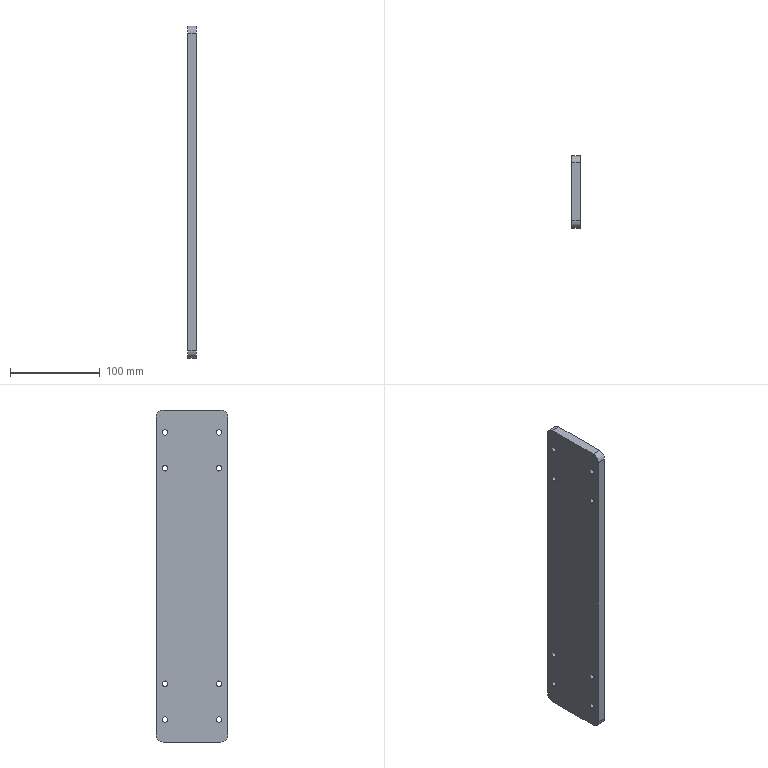Component | SolidWorks | VerticalMovingRectangularTubeWeldment-1_RectangularTubeEndPlate-2 | 1 solid | 26 faces | box 10 x 80 x 370 mm | volume 293189 mm3 | cylinder 20 | plane 6 | commonest cylinder face diameters 6 x16 16 x4 | material Plain Carbon Steel
STEP:
#1=COLOUR_RGB('',0.7922,0.8196,0.9333);
#2=FILL_AREA_STYLE_COLOUR('',#1);
#3=FILL_AREA_STYLE('',(#2));
#4=SURFACE_STYLE_FILL_AREA(#3);
#5=SURFACE_SIDE_STYLE('',(#4));
#6=SURFACE_STYLE_USAGE(.BOTH.,#5);
#7=PRESENTATION_STYLE_ASSIGNMENT((#6));
#8=CARTESIAN_POINT('',(19.685,1.181,12.913));
#9=VERTEX_POINT('',#8);
#10=CARTESIAN_POINT('',(19.685,1.181,12.677));
#11=VERTEX_POINT('',#10);
#12=CARTESIAN_POINT('',(19.685,1.181,12.795));
#13=DIRECTION('',(1.,0.,0.));
#14=DIRECTION('',(0.,1.,0.));
#15=AXIS2_PLACEMENT_3D('',#12,#13,#14);
#16=CIRCLE('',#15,0.1181);
#17=EDGE_CURVE('',#9,#11,#16,.T.);
#18=ORIENTED_EDGE('',*,*,#17,.F.);
#19=CARTESIAN_POINT('',(20.079,1.181,12.913));
#20=VERTEX_POINT('',#19);
#21=CARTESIAN_POINT('',(20.079,1.181,12.913));
#22=DIRECTION('',(1.,0.,0.));
#23=VECTOR('',#22,39.37);
#24=LINE('',#21,#23);
#25=EDGE_CURVE('',#9,#20,#24,.T.);
#26=ORIENTED_EDGE('',*,*,#25,.T.);
#27=CARTESIAN_POINT('',(20.079,1.181,12.677));
#28=VERTEX_POINT('',#27);
#29=CARTESIAN_POINT('',(20.079,1.181,12.795));
#30=DIRECTION('',(1.,0.,0.));
#31=DIRECTION('',(0.,0.,-1.));
#32=AXIS2_PLACEMENT_3D('',#29,#30,#31);
#33=CIRCLE('',#32,0.1181);
#34=EDGE_CURVE('',#20,#28,#33,.T.);
#35=ORIENTED_EDGE('',*,*,#34,.T.);
#36=CARTESIAN_POINT('',(20.079,1.181,12.677));
#37=DIRECTION('',(1.,0.,0.));
#38=VECTOR('',#37,39.37);
#39=LINE('',#36,#38);
#40=EDGE_CURVE('',#11,#28,#39,.T.);
#41=ORIENTED_EDGE('',*,*,#40,.F.);
#42=EDGE_LOOP('',(#18,#26,#35,#41));
#43=FACE_OUTER_BOUND('',#42,.T.);
#44=CARTESIAN_POINT('',(20.079,1.181,12.795));
#45=DIRECTION('',(1.,0.,0.));
#46=DIRECTION('',(0.,0.,-1.));
#47=AXIS2_PLACEMENT_3D('',#44,#45,#46);
#48=CYLINDRICAL_SURFACE('',#47,0.1181);
#49=ADVANCED_FACE('',(#43),#48,.F.);
#50=CARTESIAN_POINT('',(19.685,1.181,11.339));
#51=VERTEX_POINT('',#50);
#52=CARTESIAN_POINT('',(19.685,1.181,11.102));
#53=VERTEX_POINT('',#52);
#54=CARTESIAN_POINT('',(19.685,1.181,11.22));
#55=DIRECTION('',(1.,0.,0.));
#56=DIRECTION('',(0.,1.,0.));
#57=AXIS2_PLACEMENT_3D('',#54,#55,#56);
#58=CIRCLE('',#57,0.1181);
#59=EDGE_CURVE('',#51,#53,#58,.T.);
#60=ORIENTED_EDGE('',*,*,#59,.F.);
#61=CARTESIAN_POINT('',(20.079,1.181,11.339));
#62=VERTEX_POINT('',#61);
#63=CARTESIAN_POINT('',(20.079,1.181,11.339));
#64=DIRECTION('',(1.,0.,0.));
#65=VECTOR('',#64,39.37);
#66=LINE('',#63,#65);
#67=EDGE_CURVE('',#51,#62,#66,.T.);
#68=ORIENTED_EDGE('',*,*,#67,.T.);
#69=CARTESIAN_POINT('',(20.079,1.181,11.102));
#70=VERTEX_POINT('',#69);
#71=CARTESIAN_POINT('',(20.079,1.181,11.22));
#72=DIRECTION('',(1.,0.,0.));
#73=DIRECTION('',(0.,0.,-1.));
#74=AXIS2_PLACEMENT_3D('',#71,#72,#73);
#75=CIRCLE('',#74,0.1181);
#76=EDGE_CURVE('',#62,#70,#75,.T.);
#77=ORIENTED_EDGE('',*,*,#76,.T.);
#78=CARTESIAN_POINT('',(20.079,1.181,11.102));
#79=DIRECTION('',(1.,0.,0.));
#80=VECTOR('',#79,39.37);
#81=LINE('',#78,#80);
#82=EDGE_CURVE('',#53,#70,#81,.T.);
#83=ORIENTED_EDGE('',*,*,#82,.F.);
#84=EDGE_LOOP('',(#60,#68,#77,#83));
#85=FACE_OUTER_BOUND('',#84,.T.);
#86=CARTESIAN_POINT('',(20.079,1.181,11.22));
#87=DIRECTION('',(1.,0.,0.));
#88=DIRECTION('',(0.,0.,-1.));
#89=AXIS2_PLACEMENT_3D('',#86,#87,#88);
#90=CYLINDRICAL_SURFACE('',#89,0.1181);
#91=ADVANCED_FACE('',(#85),#90,.F.);
#92=CARTESIAN_POINT('',(19.685,1.181,1.89));
#93=VERTEX_POINT('',#92);
#94=CARTESIAN_POINT('',(19.685,1.181,1.654));
#95=VERTEX_POINT('',#94);
#96=CARTESIAN_POINT('',(19.685,1.181,1.772));
#97=DIRECTION('',(1.,0.,0.));
#98=DIRECTION('',(0.,1.,0.));
#99=AXIS2_PLACEMENT_3D('',#96,#97,#98);
#100=CIRCLE('',#99,0.1181);
#101=EDGE_CURVE('',#93,#95,#100,.T.);
#102=ORIENTED_EDGE('',*,*,#101,.F.);
#103=CARTESIAN_POINT('',(20.079,1.181,1.89));
#104=VERTEX_POINT('',#103);
#105=CARTESIAN_POINT('',(20.079,1.181,1.89));
#106=DIRECTION('',(1.,0.,0.));
#107=VECTOR('',#106,39.37);
#108=LINE('',#105,#107);
#109=EDGE_CURVE('',#93,#104,#108,.T.);
#110=ORIENTED_EDGE('',*,*,#109,.T.);
#111=CARTESIAN_POINT('',(20.079,1.181,1.654));
#112=VERTEX_POINT('',#111);
#113=CARTESIAN_POINT('',(20.079,1.181,1.772));
#114=DIRECTION('',(1.,0.,0.));
#115=DIRECTION('',(0.,0.,-1.));
#116=AXIS2_PLACEMENT_3D('',#113,#114,#115);
#117=CIRCLE('',#116,0.1181);
#118=EDGE_CURVE('',#104,#112,#117,.T.);
#119=ORIENTED_EDGE('',*,*,#118,.T.);
#120=CARTESIAN_POINT('',(20.079,1.181,1.654));
#121=DIRECTION('',(1.,0.,0.));
#122=VECTOR('',#121,39.37);
#123=LINE('',#120,#122);
#124=EDGE_CURVE('',#95,#112,#123,.T.);
#125=ORIENTED_EDGE('',*,*,#124,.F.);
#126=EDGE_LOOP('',(#102,#110,#119,#125));
#127=FACE_OUTER_BOUND('',#126,.T.);
#128=CARTESIAN_POINT('',(20.079,1.181,1.772));
#129=DIRECTION('',(1.,0.,0.));
#130=DIRECTION('',(0.,0.,-1.));
#131=AXIS2_PLACEMENT_3D('',#128,#129,#130);
#132=CYLINDRICAL_SURFACE('',#131,0.1181);
#133=ADVANCED_FACE('',(#127),#132,.F.);
#134=CARTESIAN_POINT('',(19.685,1.181,0.315));
#135=VERTEX_POINT('',#134);
#136=CARTESIAN_POINT('',(19.685,1.181,0.07874));
#137=VERTEX_POINT('',#136);
#138=CARTESIAN_POINT('',(19.685,1.181,0.1969));
#139=DIRECTION('',(1.,0.,0.));
#140=DIRECTION('',(0.,1.,-0.));
#141=AXIS2_PLACEMENT_3D('',#138,#139,#140);
#142=CIRCLE('',#141,0.1181);
#143=EDGE_CURVE('',#135,#137,#142,.T.);
#144=ORIENTED_EDGE('',*,*,#143,.F.);
#145=CARTESIAN_POINT('',(20.079,1.181,0.315));
#146=VERTEX_POINT('',#145);
#147=CARTESIAN_POINT('',(20.079,1.181,0.315));
#148=DIRECTION('',(1.,0.,0.));
#149=VECTOR('',#148,39.37);
#150=LINE('',#147,#149);
#151=EDGE_CURVE('',#135,#146,#150,.T.);
#152=ORIENTED_EDGE('',*,*,#151,.T.);
#153=CARTESIAN_POINT('',(20.079,1.181,0.07874));
#154=VERTEX_POINT('',#153);
#155=CARTESIAN_POINT('',(20.079,1.181,0.1969));
#156=DIRECTION('',(1.,0.,0.));
#157=DIRECTION('',(0.,0.,-1.));
#158=AXIS2_PLACEMENT_3D('',#155,#156,#157);
#159=CIRCLE('',#158,0.1181);
#160=EDGE_CURVE('',#146,#154,#159,.T.);
#161=ORIENTED_EDGE('',*,*,#160,.T.);
#162=CARTESIAN_POINT('',(20.079,1.181,0.07874));
#163=DIRECTION('',(1.,0.,0.));
#164=VECTOR('',#163,39.37);
#165=LINE('',#162,#164);
#166=EDGE_CURVE('',#137,#154,#165,.T.);
#167=ORIENTED_EDGE('',*,*,#166,.F.);
#168=EDGE_LOOP('',(#144,#152,#161,#167));
#169=FACE_OUTER_BOUND('',#168,.T.);
#170=CARTESIAN_POINT('',(20.079,1.181,0.1969));
#171=DIRECTION('',(1.,0.,0.));
#172=DIRECTION('',(0.,0.,-1.));
#173=AXIS2_PLACEMENT_3D('',#170,#171,#172);
#174=CYLINDRICAL_SURFACE('',#173,0.1181);
#175=ADVANCED_FACE('',(#169),#174,.F.);
#176=CARTESIAN_POINT('',(19.685,-1.181,12.913));
#177=VERTEX_POINT('',#176);
#178=CARTESIAN_POINT('',(19.685,-1.181,12.677));
#179=VERTEX_POINT('',#178);
#180=CARTESIAN_POINT('',(19.685,-1.181,12.795));
#181=DIRECTION('',(1.,0.,0.));
#182=DIRECTION('',(0.,1.,0.));
#183=AXIS2_PLACEMENT_3D('',#180,#181,#182);
#184=CIRCLE('',#183,0.1181);
#185=EDGE_CURVE('',#177,#179,#184,.T.);
#186=ORIENTED_EDGE('',*,*,#185,.F.);
#187=CARTESIAN_POINT('',(20.079,-1.181,12.913));
#188=VERTEX_POINT('',#187);
#189=CARTESIAN_POINT('',(20.079,-1.181,12.913));
#190=DIRECTION('',(1.,0.,0.));
#191=VECTOR('',#190,39.37);
#192=LINE('',#189,#191);
#193=EDGE_CURVE('',#177,#188,#192,.T.);
#194=ORIENTED_EDGE('',*,*,#193,.T.);
#195=CARTESIAN_POINT('',(20.079,-1.181,12.677));
#196=VERTEX_POINT('',#195);
#197=CARTESIAN_POINT('',(20.079,-1.181,12.795));
#198=DIRECTION('',(1.,0.,0.));
#199=DIRECTION('',(0.,0.,-1.));
#200=AXIS2_PLACEMENT_3D('',#197,#198,#199);
#201=CIRCLE('',#200,0.1181);
#202=EDGE_CURVE('',#188,#196,#201,.T.);
#203=ORIENTED_EDGE('',*,*,#202,.T.);
#204=CARTESIAN_POINT('',(20.079,-1.181,12.677));
#205=DIRECTION('',(1.,0.,0.));
#206=VECTOR('',#205,39.37);
#207=LINE('',#204,#206);
#208=EDGE_CURVE('',#179,#196,#207,.T.);
#209=ORIENTED_EDGE('',*,*,#208,.F.);
#210=EDGE_LOOP('',(#186,#194,#203,#209));
#211=FACE_OUTER_BOUND('',#210,.T.);
#212=CARTESIAN_POINT('',(20.079,-1.181,12.795));
#213=DIRECTION('',(1.,0.,0.));
#214=DIRECTION('',(0.,0.,-1.));
#215=AXIS2_PLACEMENT_3D('',#212,#213,#214);
#216=CYLINDRICAL_SURFACE('',#215,0.1181);
#217=ADVANCED_FACE('',(#211),#216,.F.);
#218=CARTESIAN_POINT('',(19.685,-1.181,11.339));
#219=VERTEX_POINT('',#218);
#220=CARTESIAN_POINT('',(19.685,-1.181,11.102));
#221=VERTEX_POINT('',#220);
#222=CARTESIAN_POINT('',(19.685,-1.181,11.22));
#223=DIRECTION('',(1.,0.,0.));
#224=DIRECTION('',(0.,1.,0.));
#225=AXIS2_PLACEMENT_3D('',#222,#223,#224);
#226=CIRCLE('',#225,0.1181);
#227=EDGE_CURVE('',#219,#221,#226,.T.);
#228=ORIENTED_EDGE('',*,*,#227,.F.);
#229=CARTESIAN_POINT('',(20.079,-1.181,11.339));
#230=VERTEX_POINT('',#229);
#231=CARTESIAN_POINT('',(20.079,-1.181,11.339));
#232=DIRECTION('',(1.,0.,0.));
#233=VECTOR('',#232,39.37);
#234=LINE('',#231,#233);
#235=EDGE_CURVE('',#219,#230,#234,.T.);
#236=ORIENTED_EDGE('',*,*,#235,.T.);
#237=CARTESIAN_POINT('',(20.079,-1.181,11.102));
#238=VERTEX_POINT('',#237);
#239=CARTESIAN_POINT('',(20.079,-1.181,11.22));
#240=DIRECTION('',(1.,0.,0.));
#241=DIRECTION('',(0.,0.,-1.));
#242=AXIS2_PLACEMENT_3D('',#239,#240,#241);
#243=CIRCLE('',#242,0.1181);
#244=EDGE_CURVE('',#230,#238,#243,.T.);
#245=ORIENTED_EDGE('',*,*,#244,.T.);
#246=CARTESIAN_POINT('',(20.079,-1.181,11.102));
#247=DIRECTION('',(1.,0.,0.));
#248=VECTOR('',#247,39.37);
#249=LINE('',#246,#248);
#250=EDGE_CURVE('',#221,#238,#249,.T.);
#251=ORIENTED_EDGE('',*,*,#250,.F.);
#252=EDGE_LOOP('',(#228,#236,#245,#251));
#253=FACE_OUTER_BOUND('',#252,.T.);
#254=CARTESIAN_POINT('',(20.079,-1.181,11.22));
#255=DIRECTION('',(1.,0.,0.));
#256=DIRECTION('',(0.,0.,-1.));
#257=AXIS2_PLACEMENT_3D('',#254,#255,#256);
#258=CYLINDRICAL_SURFACE('',#257,0.1181);
#259=ADVANCED_FACE('',(#253),#258,.F.);
#260=CARTESIAN_POINT('',(19.685,-1.181,1.89));
#261=VERTEX_POINT('',#260);
#262=CARTESIAN_POINT('',(19.685,-1.181,1.654));
#263=VERTEX_POINT('',#262);
#264=CARTESIAN_POINT('',(19.685,-1.181,1.772));
#265=DIRECTION('',(1.,0.,0.));
#266=DIRECTION('',(0.,1.,0.));
#267=AXIS2_PLACEMENT_3D('',#264,#265,#266);
#268=CIRCLE('',#267,0.1181);
#269=EDGE_CURVE('',#261,#263,#268,.T.);
#270=ORIENTED_EDGE('',*,*,#269,.F.);
#271=CARTESIAN_POINT('',(20.079,-1.181,1.89));
#272=VERTEX_POINT('',#271);
#273=CARTESIAN_POINT('',(20.079,-1.181,1.89));
#274=DIRECTION('',(1.,0.,0.));
#275=VECTOR('',#274,39.37);
#276=LINE('',#273,#275);
#277=EDGE_CURVE('',#261,#272,#276,.T.);
#278=ORIENTED_EDGE('',*,*,#277,.T.);
#279=CARTESIAN_POINT('',(20.079,-1.181,1.654));
#280=VERTEX_POINT('',#279);
#281=CARTESIAN_POINT('',(20.079,-1.181,1.772));
#282=DIRECTION('',(1.,0.,0.));
#283=DIRECTION('',(0.,0.,-1.));
#284=AXIS2_PLACEMENT_3D('',#281,#282,#283);
#285=CIRCLE('',#284,0.1181);
#286=EDGE_CURVE('',#272,#280,#285,.T.);
#287=ORIENTED_EDGE('',*,*,#286,.T.);
#288=CARTESIAN_POINT('',(20.079,-1.181,1.654));
#289=DIRECTION('',(1.,0.,0.));
#290=VECTOR('',#289,39.37);
#291=LINE('',#288,#290);
#292=EDGE_CURVE('',#263,#280,#291,.T.);
#293=ORIENTED_EDGE('',*,*,#292,.F.);
#294=EDGE_LOOP('',(#270,#278,#287,#293));
#295=FACE_OUTER_BOUND('',#294,.T.);
#296=CARTESIAN_POINT('',(20.079,-1.181,1.772));
#297=DIRECTION('',(1.,0.,0.));
#298=DIRECTION('',(0.,0.,-1.));
#299=AXIS2_PLACEMENT_3D('',#296,#297,#298);
#300=CYLINDRICAL_SURFACE('',#299,0.1181);
#301=ADVANCED_FACE('',(#295),#300,.F.);
#302=CARTESIAN_POINT('',(19.685,-1.181,0.315));
#303=VERTEX_POINT('',#302);
#304=CARTESIAN_POINT('',(19.685,-1.181,0.07874));
#305=VERTEX_POINT('',#304);
#306=CARTESIAN_POINT('',(19.685,-1.181,0.1969));
#307=DIRECTION('',(1.,0.,0.));
#308=DIRECTION('',(0.,1.,-0.));
#309=AXIS2_PLACEMENT_3D('',#306,#307,#308);
#310=CIRCLE('',#309,0.1181);
#311=EDGE_CURVE('',#303,#305,#310,.T.);
#312=ORIENTED_EDGE('',*,*,#311,.F.);
#313=CARTESIAN_POINT('',(20.079,-1.181,0.315));
#314=VERTEX_POINT('',#313);
#315=CARTESIAN_POINT('',(20.079,-1.181,0.315));
#316=DIRECTION('',(1.,0.,0.));
#317=VECTOR('',#316,39.37);
#318=LINE('',#315,#317);
#319=EDGE_CURVE('',#303,#314,#318,.T.);
#320=ORIENTED_EDGE('',*,*,#319,.T.);
#321=CARTESIAN_POINT('',(20.079,-1.181,0.07874));
#322=VERTEX_POINT('',#321);
#323=CARTESIAN_POINT('',(20.079,-1.181,0.1969));
#324=DIRECTION('',(1.,0.,0.));
#325=DIRECTION('',(0.,0.,-1.));
#326=AXIS2_PLACEMENT_3D('',#323,#324,#325);
#327=CIRCLE('',#326,0.1181);
#328=EDGE_CURVE('',#314,#322,#327,.T.);
#329=ORIENTED_EDGE('',*,*,#328,.T.);
#330=CARTESIAN_POINT('',(20.079,-1.181,0.07874));
#331=DIRECTION('',(1.,0.,0.));
#332=VECTOR('',#331,39.37);
#333=LINE('',#330,#332);
#334=EDGE_CURVE('',#305,#322,#333,.T.);
#335=ORIENTED_EDGE('',*,*,#334,.F.);
#336=EDGE_LOOP('',(#312,#320,#329,#335));
#337=FACE_OUTER_BOUND('',#336,.T.);
#338=CARTESIAN_POINT('',(20.079,-1.181,0.1969));
#339=DIRECTION('',(1.,0.,0.));
#340=DIRECTION('',(0.,0.,-1.));
#341=AXIS2_PLACEMENT_3D('',#338,#339,#340);
#342=CYLINDRICAL_SURFACE('',#341,0.1181);
#343=ADVANCED_FACE('',(#337),#342,.F.);
#344=CARTESIAN_POINT('',(20.079,1.575,-0.4724));
#345=VERTEX_POINT('',#344);
#346=CARTESIAN_POINT('',(20.079,1.575,13.465));
#347=VERTEX_POINT('',#346);
#348=CARTESIAN_POINT('',(20.079,1.575,13.78));
#349=DIRECTION('',(0.,0.,1.));
#350=VECTOR('',#349,39.37);
#351=LINE('',#348,#350);
#352=EDGE_CURVE('',#345,#347,#351,.T.);
#353=ORIENTED_EDGE('',*,*,#352,.F.);
#354=CARTESIAN_POINT('',(19.685,1.575,-0.4724));
#355=VERTEX_POINT('',#354);
#356=CARTESIAN_POINT('',(20.079,1.575,-0.4724));
#357=DIRECTION('',(-1.,0.,0.));
#358=VECTOR('',#357,39.37);
#359=LINE('',#356,#358);
#360=EDGE_CURVE('',#345,#355,#359,.T.);
#361=ORIENTED_EDGE('',*,*,#360,.T.);
#362=CARTESIAN_POINT('',(19.685,1.575,13.465));
#363=VERTEX_POINT('',#362);
#364=CARTESIAN_POINT('',(19.685,1.575,13.78));
#365=DIRECTION('',(0.,0.,1.));
#366=VECTOR('',#365,39.37);
#367=LINE('',#364,#366);
#368=EDGE_CURVE('',#355,#363,#367,.T.);
#369=ORIENTED_EDGE('',*,*,#368,.T.);
#370=CARTESIAN_POINT('',(20.079,1.575,13.465));
#371=DIRECTION('',(1.,0.,0.));
#372=VECTOR('',#371,39.37);
#373=LINE('',#370,#372);
#374=EDGE_CURVE('',#363,#347,#373,.T.);
#375=ORIENTED_EDGE('',*,*,#374,.T.);
#376=EDGE_LOOP('',(#353,#361,#369,#375));
#377=FACE_OUTER_BOUND('',#376,.T.);
#378=CARTESIAN_POINT('',(20.079,1.575,13.78));
#379=DIRECTION('',(0.,-1.,0.));
#380=DIRECTION('',(0.,-0.,-1.));
#381=AXIS2_PLACEMENT_3D('',#378,#379,#380);
#382=PLANE('',#381);
#383=ADVANCED_FACE('',(#377),#382,.F.);
#384=CARTESIAN_POINT('',(19.685,1.26,13.78));
#385=VERTEX_POINT('',#384);
#386=CARTESIAN_POINT('',(19.685,-1.26,13.78));
#387=VERTEX_POINT('',#386);
#388=CARTESIAN_POINT('',(19.685,-1.575,13.78));
#389=DIRECTION('',(0.,-1.,0.));
#390=VECTOR('',#389,39.37);
#391=LINE('',#388,#390);
#392=EDGE_CURVE('',#385,#387,#391,.T.);
#393=ORIENTED_EDGE('',*,*,#392,.T.);
#394=CARTESIAN_POINT('',(20.079,-1.26,13.78));
#395=VERTEX_POINT('',#394);
#396=CARTESIAN_POINT('',(20.079,-1.26,13.78));
#397=DIRECTION('',(1.,0.,0.));
#398=VECTOR('',#397,39.37);
#399=LINE('',#396,#398);
#400=EDGE_CURVE('',#387,#395,#399,.T.);
#401=ORIENTED_EDGE('',*,*,#400,.T.);
#402=CARTESIAN_POINT('',(20.079,1.26,13.78));
#403=VERTEX_POINT('',#402);
#404=CARTESIAN_POINT('',(20.079,-1.575,13.78));
#405=DIRECTION('',(0.,-1.,0.));
#406=VECTOR('',#405,39.37);
#407=LINE('',#404,#406);
#408=EDGE_CURVE('',#403,#395,#407,.T.);
#409=ORIENTED_EDGE('',*,*,#408,.F.);
#410=CARTESIAN_POINT('',(20.079,1.26,13.78));
#411=DIRECTION('',(-1.,0.,0.));
#412=VECTOR('',#411,39.37);
#413=LINE('',#410,#412);
#414=EDGE_CURVE('',#403,#385,#413,.T.);
#415=ORIENTED_EDGE('',*,*,#414,.T.);
#416=EDGE_LOOP('',(#393,#401,#409,#415));
#417=FACE_OUTER_BOUND('',#416,.T.);
#418=CARTESIAN_POINT('',(20.079,-1.575,13.78));
#419=DIRECTION('',(0.,-0.,-1.));
#420=DIRECTION('',(-1.,0.,0.));
#421=AXIS2_PLACEMENT_3D('',#418,#419,#420);
#422=PLANE('',#421);
#423=ADVANCED_FACE('',(#417),#422,.F.);
#424=CARTESIAN_POINT('',(19.685,-1.575,13.465));
#425=VERTEX_POINT('',#424);
#426=CARTESIAN_POINT('',(19.685,-1.575,-0.4724));
#427=VERTEX_POINT('',#426);
#428=CARTESIAN_POINT('',(19.685,-1.575,13.78));
#429=DIRECTION('',(0.,-0.,-1.));
#430=VECTOR('',#429,39.37);
#431=LINE('',#428,#430);
#432=EDGE_CURVE('',#425,#427,#431,.T.);
#433=ORIENTED_EDGE('',*,*,#432,.T.);
#434=CARTESIAN_POINT('',(20.079,-1.575,-0.4724));
#435=VERTEX_POINT('',#434);
#436=CARTESIAN_POINT('',(20.079,-1.575,-0.4724));
#437=DIRECTION('',(1.,0.,0.));
#438=VECTOR('',#437,39.37);
#439=LINE('',#436,#438);
#440=EDGE_CURVE('',#427,#435,#439,.T.);
#441=ORIENTED_EDGE('',*,*,#440,.T.);
#442=CARTESIAN_POINT('',(20.079,-1.575,13.465));
#443=VERTEX_POINT('',#442);
#444=CARTESIAN_POINT('',(20.079,-1.575,13.78));
#445=DIRECTION('',(0.,-0.,-1.));
#446=VECTOR('',#445,39.37);
#447=LINE('',#444,#446);
#448=EDGE_CURVE('',#443,#435,#447,.T.);
#449=ORIENTED_EDGE('',*,*,#448,.F.);
#450=CARTESIAN_POINT('',(20.079,-1.575,13.465));
#451=DIRECTION('',(-1.,0.,0.));
#452=VECTOR('',#451,39.37);
#453=LINE('',#450,#452);
#454=EDGE_CURVE('',#443,#425,#453,.T.);
#455=ORIENTED_EDGE('',*,*,#454,.T.);
#456=EDGE_LOOP('',(#433,#441,#449,#455));
#457=FACE_OUTER_BOUND('',#456,.T.);
#458=CARTESIAN_POINT('',(20.079,-1.575,13.78));
#459=DIRECTION('',(0.,1.,-0.));
#460=DIRECTION('',(0.,0.,1.));
#461=AXIS2_PLACEMENT_3D('',#458,#459,#460);
#462=PLANE('',#461);
#463=ADVANCED_FACE('',(#457),#462,.F.);
#464=CARTESIAN_POINT('',(20.079,-1.26,-0.7874));
#465=VERTEX_POINT('',#464);
#466=CARTESIAN_POINT('',(20.079,1.26,-0.7874));
#467=VERTEX_POINT('',#466);
#468=CARTESIAN_POINT('',(20.079,-1.575,-0.7874));
#469=DIRECTION('',(0.,1.,-0.));
#470=VECTOR('',#469,39.37);
#471=LINE('',#468,#470);
#472=EDGE_CURVE('',#465,#467,#471,.T.);
#473=ORIENTED_EDGE('',*,*,#472,.F.);
#474=CARTESIAN_POINT('',(19.685,-1.26,-0.7874));
#475=VERTEX_POINT('',#474);
#476=CARTESIAN_POINT('',(20.079,-1.26,-0.7874));
#477=DIRECTION('',(-1.,0.,0.));
#478=VECTOR('',#477,39.37);
#479=LINE('',#476,#478);
#480=EDGE_CURVE('',#465,#475,#479,.T.);
#481=ORIENTED_EDGE('',*,*,#480,.T.);
#482=CARTESIAN_POINT('',(19.685,1.26,-0.7874));
#483=VERTEX_POINT('',#482);
#484=CARTESIAN_POINT('',(19.685,-1.575,-0.7874));
#485=DIRECTION('',(0.,1.,-0.));
#486=VECTOR('',#485,39.37);
#487=LINE('',#484,#486);
#488=EDGE_CURVE('',#475,#483,#487,.T.);
#489=ORIENTED_EDGE('',*,*,#488,.T.);
#490=CARTESIAN_POINT('',(20.079,1.26,-0.7874));
#491=DIRECTION('',(1.,0.,0.));
#492=VECTOR('',#491,39.37);
#493=LINE('',#490,#492);
#494=EDGE_CURVE('',#483,#467,#493,.T.);
#495=ORIENTED_EDGE('',*,*,#494,.T.);
#496=EDGE_LOOP('',(#473,#481,#489,#495));
#497=FACE_OUTER_BOUND('',#496,.T.);
#498=CARTESIAN_POINT('',(20.079,-1.575,-0.7874));
#499=DIRECTION('',(0.,0.,1.));
#500=DIRECTION('',(1.,0.,0.));
#501=AXIS2_PLACEMENT_3D('',#498,#499,#500);
#502=PLANE('',#501);
#503=ADVANCED_FACE('',(#497),#502,.F.);
#504=CARTESIAN_POINT('',(20.079,1.181,12.795));
#505=DIRECTION('',(1.,0.,0.));
#506=DIRECTION('',(0.,0.,-1.));
#507=AXIS2_PLACEMENT_3D('',#504,#505,#506);
#508=CIRCLE('',#507,0.1181);
#509=EDGE_CURVE('',#28,#20,#508,.T.);
#510=ORIENTED_EDGE('',*,*,#509,.F.);
#511=ORIENTED_EDGE('',*,*,#34,.F.);
#512=EDGE_LOOP('',(#510,#511));
#513=FACE_BOUND('',#512,.T.);
#514=CARTESIAN_POINT('',(20.079,1.181,11.22));
#515=DIRECTION('',(1.,0.,0.));
#516=DIRECTION('',(0.,0.,-1.));
#517=AXIS2_PLACEMENT_3D('',#514,#515,#516);
#518=CIRCLE('',#517,0.1181);
#519=EDGE_CURVE('',#70,#62,#518,.T.);
#520=ORIENTED_EDGE('',*,*,#519,.F.);
#521=ORIENTED_EDGE('',*,*,#76,.F.);
#522=EDGE_LOOP('',(#520,#521));
#523=FACE_BOUND('',#522,.T.);
#524=CARTESIAN_POINT('',(20.079,1.181,1.772));
#525=DIRECTION('',(1.,0.,0.));
#526=DIRECTION('',(0.,0.,-1.));
#527=AXIS2_PLACEMENT_3D('',#524,#525,#526);
#528=CIRCLE('',#527,0.1181);
#529=EDGE_CURVE('',#112,#104,#528,.T.);
#530=ORIENTED_EDGE('',*,*,#529,.F.);
#531=ORIENTED_EDGE('',*,*,#118,.F.);
#532=EDGE_LOOP('',(#530,#531));
#533=FACE_BOUND('',#532,.T.);
#534=CARTESIAN_POINT('',(20.079,1.181,0.1969));
#535=DIRECTION('',(1.,0.,0.));
#536=DIRECTION('',(0.,0.,-1.));
#537=AXIS2_PLACEMENT_3D('',#534,#535,#536);
#538=CIRCLE('',#537,0.1181);
#539=EDGE_CURVE('',#154,#146,#538,.T.);
#540=ORIENTED_EDGE('',*,*,#539,.F.);
#541=ORIENTED_EDGE('',*,*,#160,.F.);
#542=EDGE_LOOP('',(#540,#541));
#543=FACE_BOUND('',#542,.T.);
#544=CARTESIAN_POINT('',(20.079,-1.181,12.795));
#545=DIRECTION('',(1.,0.,0.));
#546=DIRECTION('',(0.,0.,-1.));
#547=AXIS2_PLACEMENT_3D('',#544,#545,#546);
#548=CIRCLE('',#547,0.1181);
#549=EDGE_CURVE('',#196,#188,#548,.T.);
#550=ORIENTED_EDGE('',*,*,#549,.F.);
#551=ORIENTED_EDGE('',*,*,#202,.F.);
#552=EDGE_LOOP('',(#550,#551));
#553=FACE_BOUND('',#552,.T.);
#554=CARTESIAN_POINT('',(20.079,-1.181,11.22));
#555=DIRECTION('',(1.,0.,0.));
#556=DIRECTION('',(0.,0.,-1.));
#557=AXIS2_PLACEMENT_3D('',#554,#555,#556);
#558=CIRCLE('',#557,0.1181);
#559=EDGE_CURVE('',#238,#230,#558,.T.);
#560=ORIENTED_EDGE('',*,*,#559,.F.);
#561=ORIENTED_EDGE('',*,*,#244,.F.);
#562=EDGE_LOOP('',(#560,#561));
#563=FACE_BOUND('',#562,.T.);
#564=CARTESIAN_POINT('',(20.079,-1.181,1.772));
#565=DIRECTION('',(1.,0.,0.));
#566=DIRECTION('',(0.,0.,-1.));
#567=AXIS2_PLACEMENT_3D('',#564,#565,#566);
#568=CIRCLE('',#567,0.1181);
#569=EDGE_CURVE('',#280,#272,#568,.T.);
#570=ORIENTED_EDGE('',*,*,#569,.F.);
#571=ORIENTED_EDGE('',*,*,#286,.F.);
#572=EDGE_LOOP('',(#570,#571));
#573=FACE_BOUND('',#572,.T.);
#574=CARTESIAN_POINT('',(20.079,-1.181,0.1969));
#575=DIRECTION('',(1.,0.,0.));
#576=DIRECTION('',(0.,0.,-1.));
#577=AXIS2_PLACEMENT_3D('',#574,#575,#576);
#578=CIRCLE('',#577,0.1181);
#579=EDGE_CURVE('',#322,#314,#578,.T.);
#580=ORIENTED_EDGE('',*,*,#579,.F.);
#581=ORIENTED_EDGE('',*,*,#328,.F.);
#582=EDGE_LOOP('',(#580,#581));
#583=FACE_BOUND('',#582,.T.);
#584=ORIENTED_EDGE('',*,*,#448,.T.);
#585=CARTESIAN_POINT('',(20.079,-1.26,-0.4724));
#586=DIRECTION('',(1.,0.,0.));
#587=DIRECTION('',(0.,1.,-0.));
#588=AXIS2_PLACEMENT_3D('',#585,#586,#587);
#589=CIRCLE('',#588,0.315);
#590=EDGE_CURVE('',#435,#465,#589,.T.);
#591=ORIENTED_EDGE('',*,*,#590,.T.);
#592=ORIENTED_EDGE('',*,*,#472,.T.);
#593=CARTESIAN_POINT('',(20.079,1.26,-0.4724));
#594=DIRECTION('',(1.,0.,0.));
#595=DIRECTION('',(0.,1.,-0.));
#596=AXIS2_PLACEMENT_3D('',#593,#594,#595);
#597=CIRCLE('',#596,0.315);
#598=EDGE_CURVE('',#467,#345,#597,.T.);
#599=ORIENTED_EDGE('',*,*,#598,.T.);
#600=ORIENTED_EDGE('',*,*,#352,.T.);
#601=CARTESIAN_POINT('',(20.079,1.26,13.465));
#602=DIRECTION('',(1.,0.,0.));
#603=DIRECTION('',(0.,1.,0.));
#604=AXIS2_PLACEMENT_3D('',#601,#602,#603);
#605=CIRCLE('',#604,0.315);
#606=EDGE_CURVE('',#347,#403,#605,.T.);
#607=ORIENTED_EDGE('',*,*,#606,.T.);
#608=ORIENTED_EDGE('',*,*,#408,.T.);
#609=CARTESIAN_POINT('',(20.079,-1.26,13.465));
#610=DIRECTION('',(1.,0.,0.));
#611=DIRECTION('',(0.,1.,0.));
#612=AXIS2_PLACEMENT_3D('',#609,#610,#611);
#613=CIRCLE('',#612,0.315);
#614=EDGE_CURVE('',#395,#443,#613,.T.);
#615=ORIENTED_EDGE('',*,*,#614,.T.);
#616=EDGE_LOOP('',(#584,#591,#592,#599,#600,#607,#608,#615));
#617=FACE_OUTER_BOUND('',#616,.T.);
#618=CARTESIAN_POINT('',(20.079,0.,6.496));
#619=DIRECTION('',(1.,0.,0.));
#620=DIRECTION('',(0.,1.,-0.));
#621=AXIS2_PLACEMENT_3D('',#618,#619,#620);
#622=PLANE('',#621);
#623=ADVANCED_FACE('',(#513,#523,#533,#543,#553,#563,#573,#583,#617),#622,.T.);
#624=CARTESIAN_POINT('',(19.685,1.181,12.795));
#625=DIRECTION('',(1.,0.,0.));
#626=DIRECTION('',(0.,1.,0.));
#627=AXIS2_PLACEMENT_3D('',#624,#625,#626);
#628=CIRCLE('',#627,0.1181);
#629=EDGE_CURVE('',#11,#9,#628,.T.);
#630=ORIENTED_EDGE('',*,*,#629,.T.);
#631=ORIENTED_EDGE('',*,*,#17,.T.);
#632=EDGE_LOOP('',(#630,#631));
#633=FACE_BOUND('',#632,.T.);
#634=CARTESIAN_POINT('',(19.685,1.181,11.22));
#635=DIRECTION('',(1.,0.,0.));
#636=DIRECTION('',(0.,1.,0.));
#637=AXIS2_PLACEMENT_3D('',#634,#635,#636);
#638=CIRCLE('',#637,0.1181);
#639=EDGE_CURVE('',#53,#51,#638,.T.);
#640=ORIENTED_EDGE('',*,*,#639,.T.);
#641=ORIENTED_EDGE('',*,*,#59,.T.);
#642=EDGE_LOOP('',(#640,#641));
#643=FACE_BOUND('',#642,.T.);
#644=CARTESIAN_POINT('',(19.685,1.181,1.772));
#645=DIRECTION('',(1.,0.,0.));
#646=DIRECTION('',(0.,1.,0.));
#647=AXIS2_PLACEMENT_3D('',#644,#645,#646);
#648=CIRCLE('',#647,0.1181);
#649=EDGE_CURVE('',#95,#93,#648,.T.);
#650=ORIENTED_EDGE('',*,*,#649,.T.);
#651=ORIENTED_EDGE('',*,*,#101,.T.);
#652=EDGE_LOOP('',(#650,#651));
#653=FACE_BOUND('',#652,.T.);
#654=CARTESIAN_POINT('',(19.685,1.181,0.1969));
#655=DIRECTION('',(1.,0.,0.));
#656=DIRECTION('',(0.,1.,-0.));
#657=AXIS2_PLACEMENT_3D('',#654,#655,#656);
#658=CIRCLE('',#657,0.1181);
#659=EDGE_CURVE('',#137,#135,#658,.T.);
#660=ORIENTED_EDGE('',*,*,#659,.T.);
#661=ORIENTED_EDGE('',*,*,#143,.T.);
#662=EDGE_LOOP('',(#660,#661));
#663=FACE_BOUND('',#662,.T.);
#664=CARTESIAN_POINT('',(19.685,-1.181,12.795));
#665=DIRECTION('',(1.,0.,0.));
#666=DIRECTION('',(0.,1.,0.));
#667=AXIS2_PLACEMENT_3D('',#664,#665,#666);
#668=CIRCLE('',#667,0.1181);
#669=EDGE_CURVE('',#179,#177,#668,.T.);
#670=ORIENTED_EDGE('',*,*,#669,.T.);
#671=ORIENTED_EDGE('',*,*,#185,.T.);
#672=EDGE_LOOP('',(#670,#671));
#673=FACE_BOUND('',#672,.T.);
#674=CARTESIAN_POINT('',(19.685,-1.181,11.22));
#675=DIRECTION('',(1.,0.,0.));
#676=DIRECTION('',(0.,1.,0.));
#677=AXIS2_PLACEMENT_3D('',#674,#675,#676);
#678=CIRCLE('',#677,0.1181);
#679=EDGE_CURVE('',#221,#219,#678,.T.);
#680=ORIENTED_EDGE('',*,*,#679,.T.);
#681=ORIENTED_EDGE('',*,*,#227,.T.);
#682=EDGE_LOOP('',(#680,#681));
#683=FACE_BOUND('',#682,.T.);
#684=CARTESIAN_POINT('',(19.685,-1.181,1.772));
#685=DIRECTION('',(1.,0.,0.));
#686=DIRECTION('',(0.,1.,0.));
#687=AXIS2_PLACEMENT_3D('',#684,#685,#686);
#688=CIRCLE('',#687,0.1181);
#689=EDGE_CURVE('',#263,#261,#688,.T.);
#690=ORIENTED_EDGE('',*,*,#689,.T.);
#691=ORIENTED_EDGE('',*,*,#269,.T.);
#692=EDGE_LOOP('',(#690,#691));
#693=FACE_BOUND('',#692,.T.);
#694=CARTESIAN_POINT('',(19.685,-1.181,0.1969));
#695=DIRECTION('',(1.,0.,0.));
#696=DIRECTION('',(0.,1.,-0.));
#697=AXIS2_PLACEMENT_3D('',#694,#695,#696);
#698=CIRCLE('',#697,0.1181);
#699=EDGE_CURVE('',#305,#303,#698,.T.);
#700=ORIENTED_EDGE('',*,*,#699,.T.);
#701=ORIENTED_EDGE('',*,*,#311,.T.);
#702=EDGE_LOOP('',(#700,#701));
#703=FACE_BOUND('',#702,.T.);
#704=ORIENTED_EDGE('',*,*,#488,.F.);
#705=CARTESIAN_POINT('',(19.685,-1.26,-0.4724));
#706=DIRECTION('',(-1.,0.,0.));
#707=DIRECTION('',(0.,1.,-0.));
#708=AXIS2_PLACEMENT_3D('',#705,#706,#707);
#709=CIRCLE('',#708,0.315);
#710=EDGE_CURVE('',#475,#427,#709,.T.);
#711=ORIENTED_EDGE('',*,*,#710,.T.);
#712=ORIENTED_EDGE('',*,*,#432,.F.);
#713=CARTESIAN_POINT('',(19.685,-1.26,13.465));
#714=DIRECTION('',(-1.,0.,0.));
#715=DIRECTION('',(0.,1.,0.));
#716=AXIS2_PLACEMENT_3D('',#713,#714,#715);
#717=CIRCLE('',#716,0.315);
#718=EDGE_CURVE('',#425,#387,#717,.T.);
#719=ORIENTED_EDGE('',*,*,#718,.T.);
#720=ORIENTED_EDGE('',*,*,#392,.F.);
#721=CARTESIAN_POINT('',(19.685,1.26,13.465));
#722=DIRECTION('',(-1.,0.,0.));
#723=DIRECTION('',(0.,1.,0.));
#724=AXIS2_PLACEMENT_3D('',#721,#722,#723);
#725=CIRCLE('',#724,0.315);
#726=EDGE_CURVE('',#385,#363,#725,.T.);
#727=ORIENTED_EDGE('',*,*,#726,.T.);
#728=ORIENTED_EDGE('',*,*,#368,.F.);
#729=CARTESIAN_POINT('',(19.685,1.26,-0.4724));
#730=DIRECTION('',(-1.,0.,0.));
#731=DIRECTION('',(0.,1.,-0.));
#732=AXIS2_PLACEMENT_3D('',#729,#730,#731);
#733=CIRCLE('',#732,0.315);
#734=EDGE_CURVE('',#355,#483,#733,.T.);
#735=ORIENTED_EDGE('',*,*,#734,.T.);
#736=EDGE_LOOP('',(#704,#711,#712,#719,#720,#727,#728,#735));
#737=FACE_OUTER_BOUND('',#736,.T.);
#738=CARTESIAN_POINT('',(19.685,0.,6.496));
#739=DIRECTION('',(1.,0.,0.));
#740=DIRECTION('',(0.,1.,-0.));
#741=AXIS2_PLACEMENT_3D('',#738,#739,#740);
#742=PLANE('',#741);
#743=ADVANCED_FACE('',(#633,#643,#653,#663,#673,#683,#693,#703,#737),#742,.F.);
#744=ORIENTED_EDGE('',*,*,#590,.F.);
#745=ORIENTED_EDGE('',*,*,#440,.F.);
#746=ORIENTED_EDGE('',*,*,#710,.F.);
#747=ORIENTED_EDGE('',*,*,#480,.F.);
#748=EDGE_LOOP('',(#744,#745,#746,#747));
#749=FACE_OUTER_BOUND('',#748,.T.);
#750=CARTESIAN_POINT('',(20.079,-1.26,-0.4724));
#751=DIRECTION('',(-1.,0.,0.));
#752=DIRECTION('',(0.,-1.,0.));
#753=AXIS2_PLACEMENT_3D('',#750,#751,#752);
#754=CYLINDRICAL_SURFACE('',#753,0.315);
#755=ADVANCED_FACE('',(#749),#754,.T.);
#756=ORIENTED_EDGE('',*,*,#598,.F.);
#757=ORIENTED_EDGE('',*,*,#494,.F.);
#758=ORIENTED_EDGE('',*,*,#734,.F.);
#759=ORIENTED_EDGE('',*,*,#360,.F.);
#760=EDGE_LOOP('',(#756,#757,#758,#759));
#761=FACE_OUTER_BOUND('',#760,.T.);
#762=CARTESIAN_POINT('',(20.079,1.26,-0.4724));
#763=DIRECTION('',(-1.,0.,0.));
#764=DIRECTION('',(0.,-1.,0.));
#765=AXIS2_PLACEMENT_3D('',#762,#763,#764);
#766=CYLINDRICAL_SURFACE('',#765,0.315);
#767=ADVANCED_FACE('',(#761),#766,.T.);
#768=ORIENTED_EDGE('',*,*,#614,.F.);
#769=ORIENTED_EDGE('',*,*,#400,.F.);
#770=ORIENTED_EDGE('',*,*,#718,.F.);
#771=ORIENTED_EDGE('',*,*,#454,.F.);
#772=EDGE_LOOP('',(#768,#769,#770,#771));
#773=FACE_OUTER_BOUND('',#772,.T.);
#774=CARTESIAN_POINT('',(20.079,-1.26,13.465));
#775=DIRECTION('',(-1.,0.,0.));
#776=DIRECTION('',(0.,-1.,0.));
#777=AXIS2_PLACEMENT_3D('',#774,#775,#776);
#778=CYLINDRICAL_SURFACE('',#777,0.315);
#779=ADVANCED_FACE('',(#773),#778,.T.);
#780=ORIENTED_EDGE('',*,*,#606,.F.);
#781=ORIENTED_EDGE('',*,*,#374,.F.);
#782=ORIENTED_EDGE('',*,*,#726,.F.);
#783=ORIENTED_EDGE('',*,*,#414,.F.);
#784=EDGE_LOOP('',(#780,#781,#782,#783));
#785=FACE_OUTER_BOUND('',#784,.T.);
#786=CARTESIAN_POINT('',(20.079,1.26,13.465));
#787=DIRECTION('',(-1.,0.,0.));
#788=DIRECTION('',(0.,-1.,0.));
#789=AXIS2_PLACEMENT_3D('',#786,#787,#788);
#790=CYLINDRICAL_SURFACE('',#789,0.315);
#791=ADVANCED_FACE('',(#785),#790,.T.);
#792=ORIENTED_EDGE('',*,*,#319,.F.);
#793=ORIENTED_EDGE('',*,*,#699,.F.);
#794=ORIENTED_EDGE('',*,*,#334,.T.);
#795=ORIENTED_EDGE('',*,*,#579,.T.);
#796=EDGE_LOOP('',(#792,#793,#794,#795));
#797=FACE_OUTER_BOUND('',#796,.T.);
#798=CARTESIAN_POINT('',(20.079,-1.181,0.1969));
#799=DIRECTION('',(1.,0.,0.));
#800=DIRECTION('',(0.,0.,-1.));
#801=AXIS2_PLACEMENT_3D('',#798,#799,#800);
#802=CYLINDRICAL_SURFACE('',#801,0.1181);
#803=ADVANCED_FACE('',(#797),#802,.F.);
#804=ORIENTED_EDGE('',*,*,#277,.F.);
#805=ORIENTED_EDGE('',*,*,#689,.F.);
#806=ORIENTED_EDGE('',*,*,#292,.T.);
#807=ORIENTED_EDGE('',*,*,#569,.T.);
#808=EDGE_LOOP('',(#804,#805,#806,#807));
#809=FACE_OUTER_BOUND('',#808,.T.);
#810=CARTESIAN_POINT('',(20.079,-1.181,1.772));
#811=DIRECTION('',(1.,0.,0.));
#812=DIRECTION('',(0.,0.,-1.));
#813=AXIS2_PLACEMENT_3D('',#810,#811,#812);
#814=CYLINDRICAL_SURFACE('',#813,0.1181);
#815=ADVANCED_FACE('',(#809),#814,.F.);
#816=ORIENTED_EDGE('',*,*,#235,.F.);
#817=ORIENTED_EDGE('',*,*,#679,.F.);
#818=ORIENTED_EDGE('',*,*,#250,.T.);
#819=ORIENTED_EDGE('',*,*,#559,.T.);
#820=EDGE_LOOP('',(#816,#817,#818,#819));
#821=FACE_OUTER_BOUND('',#820,.T.);
#822=CARTESIAN_POINT('',(20.079,-1.181,11.22));
#823=DIRECTION('',(1.,0.,0.));
#824=DIRECTION('',(0.,0.,-1.));
#825=AXIS2_PLACEMENT_3D('',#822,#823,#824);
#826=CYLINDRICAL_SURFACE('',#825,0.1181);
#827=ADVANCED_FACE('',(#821),#826,.F.);
#828=ORIENTED_EDGE('',*,*,#193,.F.);
#829=ORIENTED_EDGE('',*,*,#669,.F.);
#830=ORIENTED_EDGE('',*,*,#208,.T.);
#831=ORIENTED_EDGE('',*,*,#549,.T.);
#832=EDGE_LOOP('',(#828,#829,#830,#831));
#833=FACE_OUTER_BOUND('',#832,.T.);
#834=CARTESIAN_POINT('',(20.079,-1.181,12.795));
#835=DIRECTION('',(1.,0.,0.));
#836=DIRECTION('',(0.,0.,-1.));
#837=AXIS2_PLACEMENT_3D('',#834,#835,#836);
#838=CYLINDRICAL_SURFACE('',#837,0.1181);
#839=ADVANCED_FACE('',(#833),#838,.F.);
#840=ORIENTED_EDGE('',*,*,#151,.F.);
#841=ORIENTED_EDGE('',*,*,#659,.F.);
#842=ORIENTED_EDGE('',*,*,#166,.T.);
#843=ORIENTED_EDGE('',*,*,#539,.T.);
#844=EDGE_LOOP('',(#840,#841,#842,#843));
#845=FACE_OUTER_BOUND('',#844,.T.);
#846=CARTESIAN_POINT('',(20.079,1.181,0.1969));
#847=DIRECTION('',(1.,0.,0.));
#848=DIRECTION('',(0.,0.,-1.));
#849=AXIS2_PLACEMENT_3D('',#846,#847,#848);
#850=CYLINDRICAL_SURFACE('',#849,0.1181);
#851=ADVANCED_FACE('',(#845),#850,.F.);
#852=ORIENTED_EDGE('',*,*,#109,.F.);
#853=ORIENTED_EDGE('',*,*,#649,.F.);
#854=ORIENTED_EDGE('',*,*,#124,.T.);
#855=ORIENTED_EDGE('',*,*,#529,.T.);
#856=EDGE_LOOP('',(#852,#853,#854,#855));
#857=FACE_OUTER_BOUND('',#856,.T.);
#858=CARTESIAN_POINT('',(20.079,1.181,1.772));
#859=DIRECTION('',(1.,0.,0.));
#860=DIRECTION('',(0.,0.,-1.));
#861=AXIS2_PLACEMENT_3D('',#858,#859,#860);
#862=CYLINDRICAL_SURFACE('',#861,0.1181);
#863=ADVANCED_FACE('',(#857),#862,.F.);
#864=ORIENTED_EDGE('',*,*,#67,.F.);
#865=ORIENTED_EDGE('',*,*,#639,.F.);
#866=ORIENTED_EDGE('',*,*,#82,.T.);
#867=ORIENTED_EDGE('',*,*,#519,.T.);
#868=EDGE_LOOP('',(#864,#865,#866,#867));
#869=FACE_OUTER_BOUND('',#868,.T.);
#870=CARTESIAN_POINT('',(20.079,1.181,11.22));
#871=DIRECTION('',(1.,0.,0.));
#872=DIRECTION('',(0.,0.,-1.));
#873=AXIS2_PLACEMENT_3D('',#870,#871,#872);
#874=CYLINDRICAL_SURFACE('',#873,0.1181);
#875=ADVANCED_FACE('',(#869),#874,.F.);
#876=ORIENTED_EDGE('',*,*,#25,.F.);
#877=ORIENTED_EDGE('',*,*,#629,.F.);
#878=ORIENTED_EDGE('',*,*,#40,.T.);
#879=ORIENTED_EDGE('',*,*,#509,.T.);
#880=EDGE_LOOP('',(#876,#877,#878,#879));
#881=FACE_OUTER_BOUND('',#880,.T.);
#882=CARTESIAN_POINT('',(20.079,1.181,12.795));
#883=DIRECTION('',(1.,0.,0.));
#884=DIRECTION('',(0.,0.,-1.));
#885=AXIS2_PLACEMENT_3D('',#882,#883,#884);
#886=CYLINDRICAL_SURFACE('',#885,0.1181);
#887=ADVANCED_FACE('',(#881),#886,.F.);
#888=CLOSED_SHELL('',(#49,#91,#133,#175,#217,#259,#301,#343,#383,#423,#463,#503,#623,#743,#755,#767,#779,#791,#803,#815,#827,#839,#851,#863,#875,#887));
#889=MANIFOLD_SOLID_BREP('',#888);
#890=STYLED_ITEM('',(#7),#889);
#891=PRESENTATION_LAYER_ASSIGNMENT('','',(#890));
#892=CARTESIAN_POINT('',(0.,0.,0.));
#893=DIRECTION('',(0.,0.,1.));
#894=DIRECTION('',(1.,0.,0.));
#895=AXIS2_PLACEMENT_3D('',#892,#893,#894);
#896=(LENGTH_UNIT()NAMED_UNIT(*)SI_UNIT($,.METRE.));
#897=LENGTH_MEASURE_WITH_UNIT(LENGTH_MEASURE(0.0254),#896);
#898=DIMENSIONAL_EXPONENTS(1.,0.,0.,0.,0.,0.,0.);
#899=(CONVERSION_BASED_UNIT('',#897)LENGTH_UNIT()NAMED_UNIT(#898));
#900=UNCERTAINTY_MEASURE_WITH_UNIT(LENGTH_MEASURE(0.00001),#899,'','');
#901=(NAMED_UNIT(*)PLANE_ANGLE_UNIT()SI_UNIT($,.RADIAN.));
#902=(NAMED_UNIT(*)SI_UNIT($,.STERADIAN.)SOLID_ANGLE_UNIT());
#903=(GEOMETRIC_REPRESENTATION_CONTEXT(3)GLOBAL_UNCERTAINTY_ASSIGNED_CONTEXT((#900))GLOBAL_UNIT_ASSIGNED_CONTEXT((#899,#901,#902))REPRESENTATION_CONTEXT('',''));
#904=ADVANCED_BREP_SHAPE_REPRESENTATION('',(#889,#895),#903);
#905=(LENGTH_UNIT()NAMED_UNIT(*)SI_UNIT($,.METRE.));
#906=LENGTH_MEASURE_WITH_UNIT(LENGTH_MEASURE(0.0254),#905);
#907=DIMENSIONAL_EXPONENTS(1.,0.,0.,0.,0.,0.,0.);
#908=(CONVERSION_BASED_UNIT('',#906)LENGTH_UNIT()NAMED_UNIT(#907));
#909=UNCERTAINTY_MEASURE_WITH_UNIT(LENGTH_MEASURE(0.00001),#908,'','');
#910=(NAMED_UNIT(*)PLANE_ANGLE_UNIT()SI_UNIT($,.RADIAN.));
#911=(NAMED_UNIT(*)SI_UNIT($,.STERADIAN.)SOLID_ANGLE_UNIT());
#912=(GEOMETRIC_REPRESENTATION_CONTEXT(3)GLOBAL_UNCERTAINTY_ASSIGNED_CONTEXT((#909))GLOBAL_UNIT_ASSIGNED_CONTEXT((#908,#910,#911))REPRESENTATION_CONTEXT('',''));
#913=MECHANICAL_DESIGN_GEOMETRIC_PRESENTATION_REPRESENTATION('',(#890),#912);